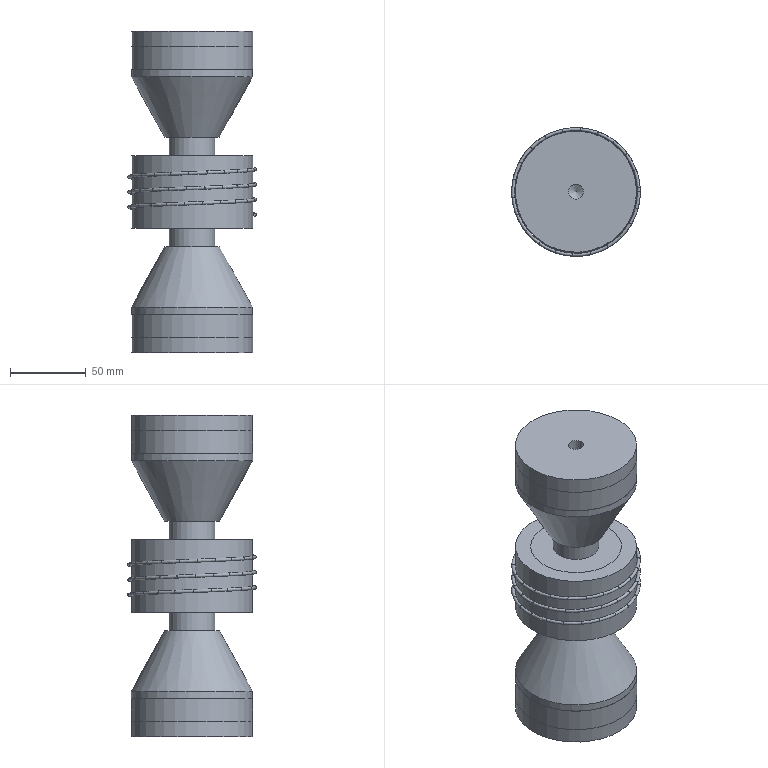Assembly | NX | mm | 12 component files | 12 solids | 123 faces | box 85 x 85 x 212 mm | volume 768635 mm3 | torus 66 | plane 26 | cylinder 25 | cone 6 | commonest cylinder face diameters 10 x8 80 x7 30 x6 60 x2 4 x2
Bill of materials:
CH3404.10-2 | 2 |  | Solid right circular cylinder, height somewhat greater than diameter, with a small central axial hole that appears blind with a conical (drill-point-like) bottom.
CH3404.10-1 | 2 |  | Truncated cone (frustum) with a short cylindrical rim at the wide end, a small central axial through hole in the wide flat face, and one small radial hole through the conical side wall.
CH3404.10-4 | 1 |  | Thin-walled cylindrical ring or short tube with a large concentric through bore; length shorter than outer diameter.
CH3404.10-7 | 2 |  | Flat circular disc with a small central through hole; thickness small relative to diameter.
CH3404.10-8 | 1 |  | Solid flat circular disc (short cylinder) with no visible holes or features.
CH3404.10-3 | 1 |  | Thick-walled cylindrical tube/bushing-like shape with a concentric through bore of roughly half the outer diameter; length slightly greater than outer diameter.
CH3404.10-5 | 1 |  | Open helical coil of round-section wire with about three turns, constant diameter and pitch, and plain cut ends.
CH3404.10-6 | 2 |  | Thin flat circular disc with a small central through hole; thinner than a similar holed disc in this set.
Mates:
1. touch align | CH3404_10-6 2 | assembly datumplane
2. touch align | CH3404_10-6 2 | assembly datumplane
3. touch align | CH3404_10-6 2 face | assembly datumaxis
4. touch align | CH3404_10-7 2 face | CH3404_10-6 2 face
5. touch align | CH3404_10-7 2 | assembly datumplane
6. touch align | CH3404_10-7 2 face | assembly datumaxis
7. touch align | CH3404_10-1 2 face | CH3404_10-7 2 face
8. touch align | CH3404_10-1 2 | CH3404_10-7 2
9. touch align | CH3404_10-1 2 face | assembly datumaxis
10. touch align | CH3404_10-2 2 face | CH3404_10-1 2 face
11. touch align | CH3404_10-2 2 | assembly datumplane
12. touch align | CH3404_10-2 2 face | assembly datumaxis
13. touch align | CH3404_10-8 1 face | CH3404_10-2 2 face
14. touch align | CH3404_10-8 1 | assembly datumplane
15. touch align | CH3404_10-8 1 face | assembly datumaxis
16. touch align | CH3404_10-3 1 datumplane | CH3404_10-8 1
17. touch align | CH3404_10-3 1 datumplane | CH3404_10-8 1
18. touch align | CH3404_10-3 1 face | assembly datumaxis
19. touch align | CH3404_10-4 1 | CH3404_10-3 1 datumplane
20. touch align | CH3404_10-4 1 | CH3404_10-3 1 datumplane
21. touch align | CH3404_10-4 1 face | assembly datumaxis
22. distance | CH3404_10-5 1 | CH3404_10-8 1
23. touch align | CH3404_10-5 1 | assembly datumplane
24. touch align | CH3404_10-5 1 | assembly datumaxis
25. touch align | CH3404_10-2 1 face | CH3404_10-8 1 face
26. touch align | CH3404_10-2 1 | assembly datumplane
27. touch align | CH3404_10-2 1 face | assembly datumaxis
28. touch align | CH3404_10-1 1 | assembly datumplane
29. touch align | CH3404_10-1 1 face | CH3404_10-2 1 face
30. touch align | CH3404_10-1 1 face | assembly datumaxis
31. touch align | CH3404_10-7 1 | assembly datumplane
32. touch align | CH3404_10-7 1 face | CH3404_10-1 1 face
33. touch align | CH3404_10-7 1 face | assembly datumaxis
34. touch align | CH3404_10-6 1 | assembly datumplane
35. touch align | CH3404_10-6 1 face | CH3404_10-7 1 face
36. touch align | CH3404_10-6 1 face | assembly datumaxis